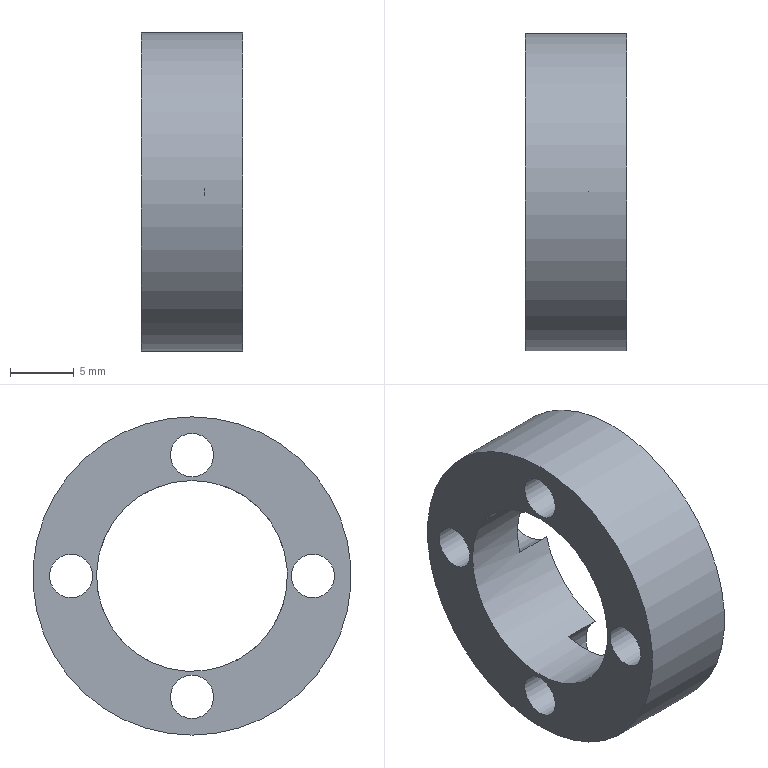Component | NX | SPACER_SLEEVE_2 | 1 solid | 16 faces | volume 2042 mm3 | cylinder 10 | plane 6 | commonest cylinder face diameters 5.8 x4 3.4 x4 25 x1 15 x1